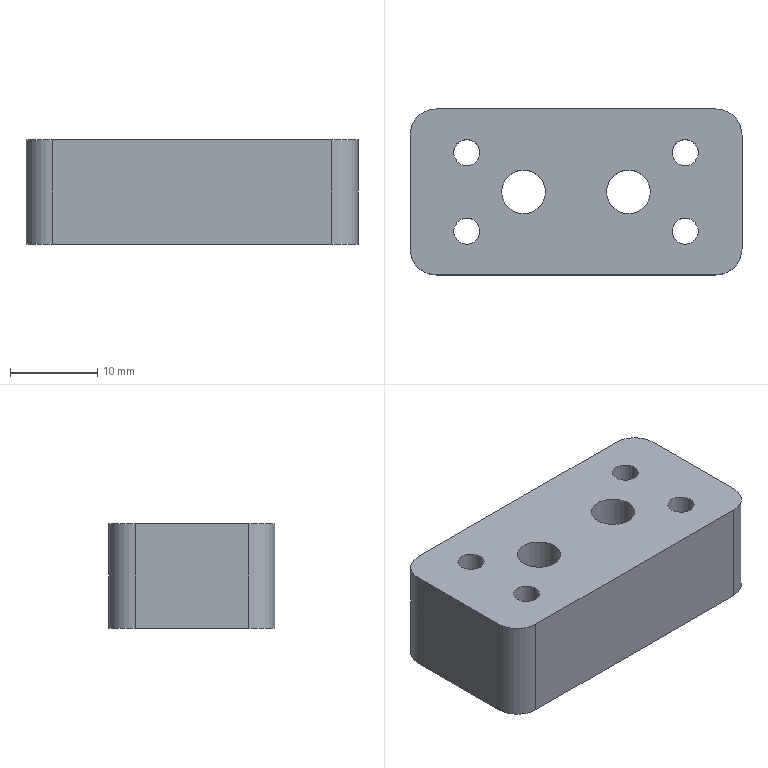Component | NX | PISTON_CYLINDER_LINK_PLATFORM | 1 solid | 16 faces | volume 7761 mm3 | cylinder 10 | plane 6 | commonest cylinder face diameters 3 x4 6 x4 5 x2